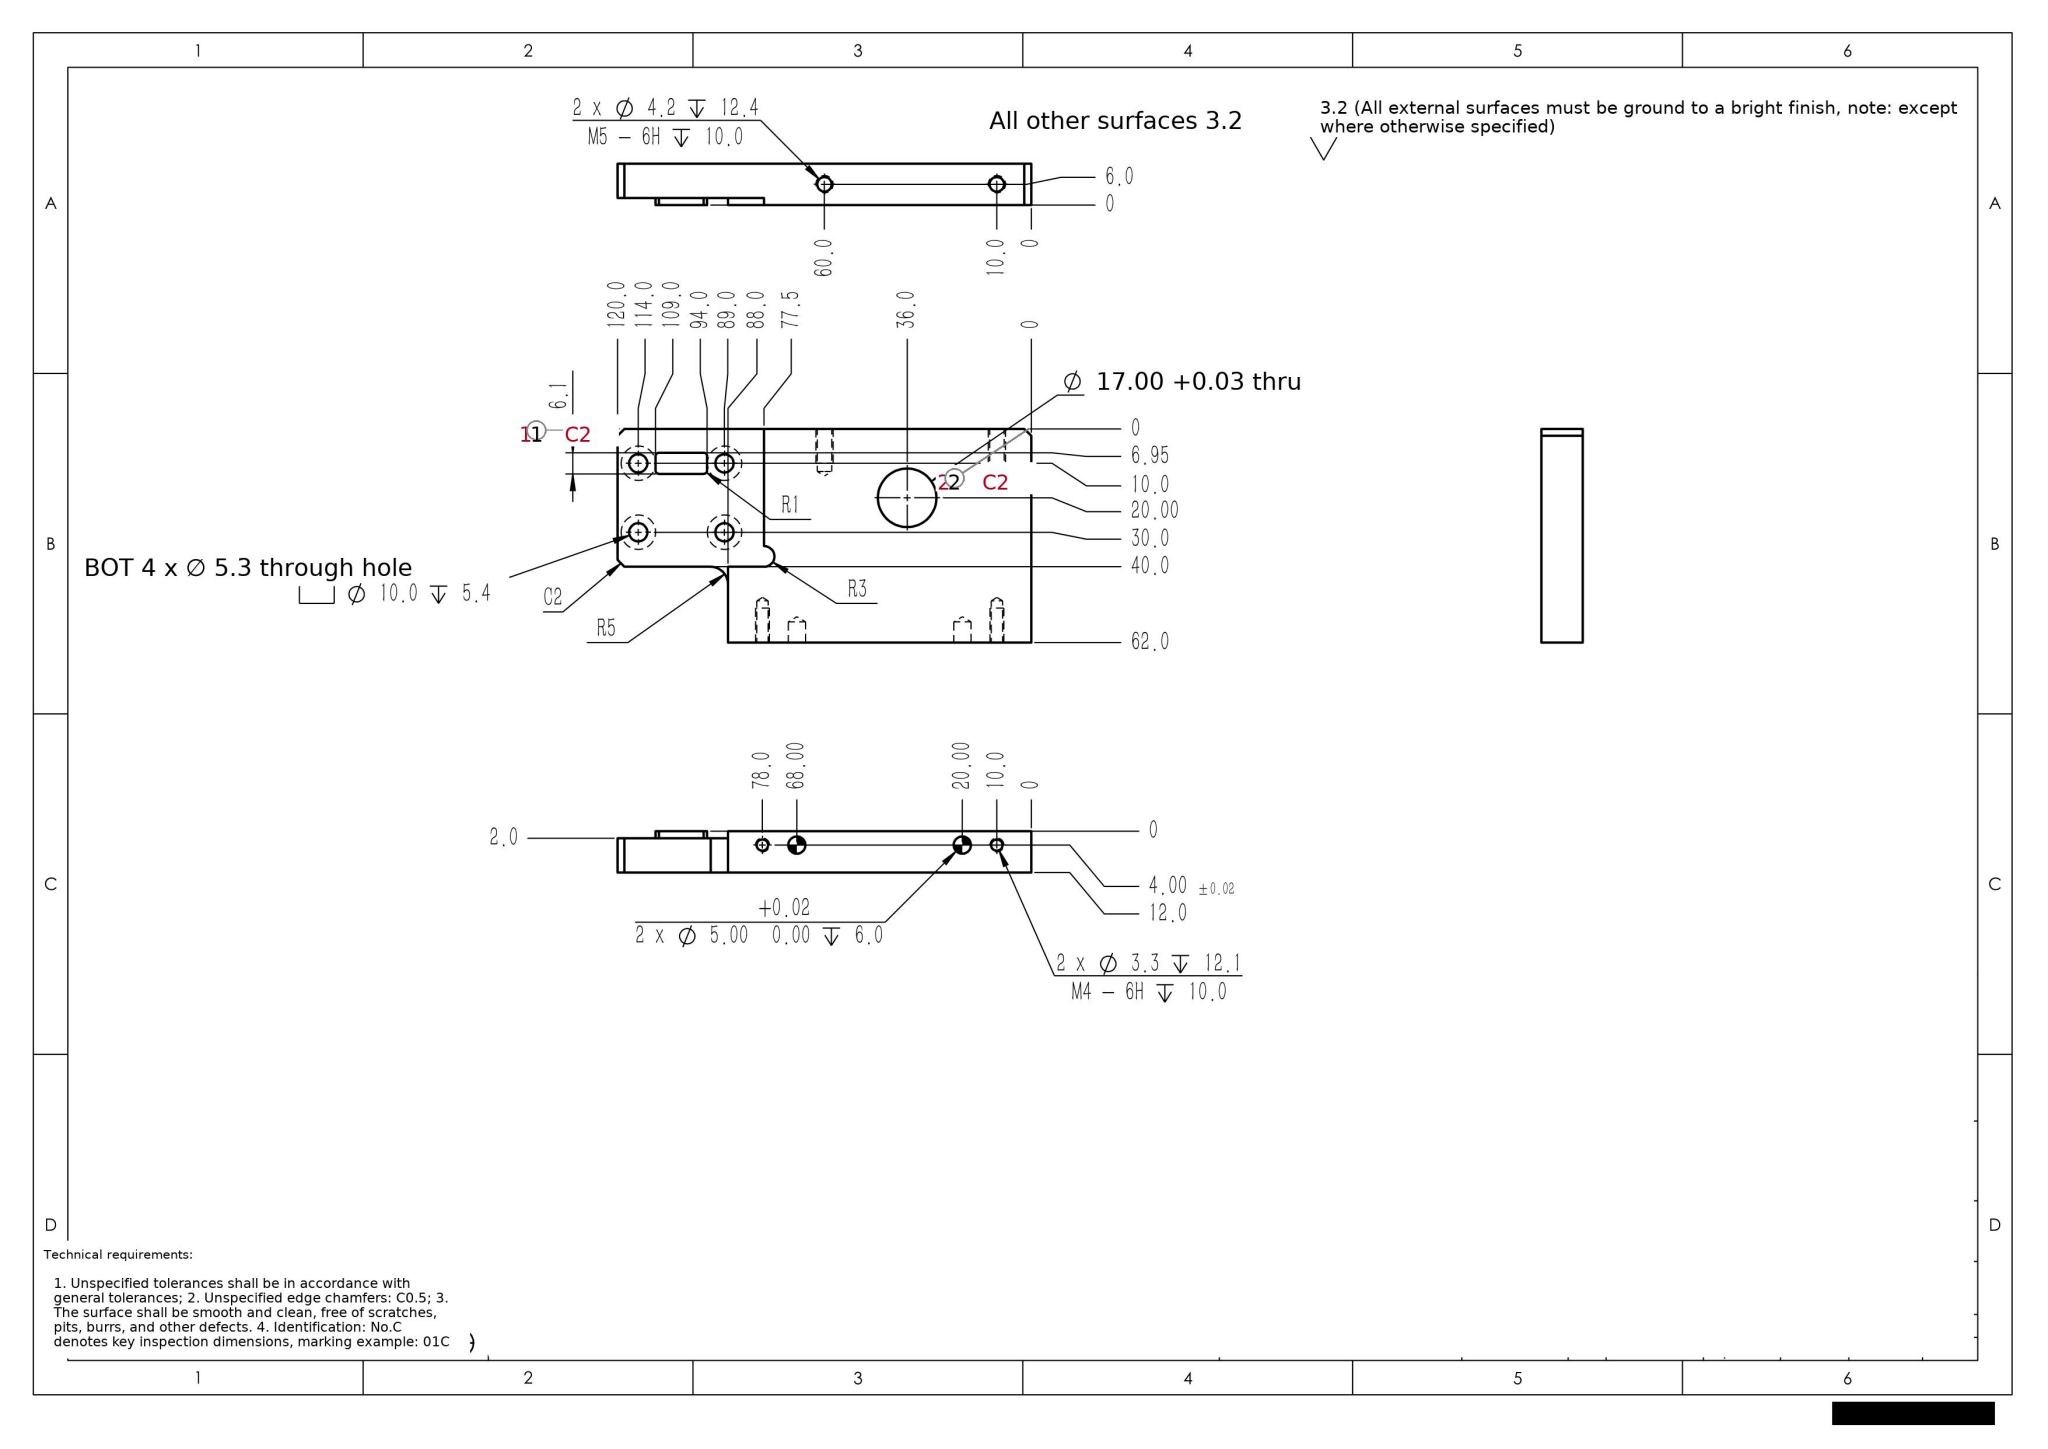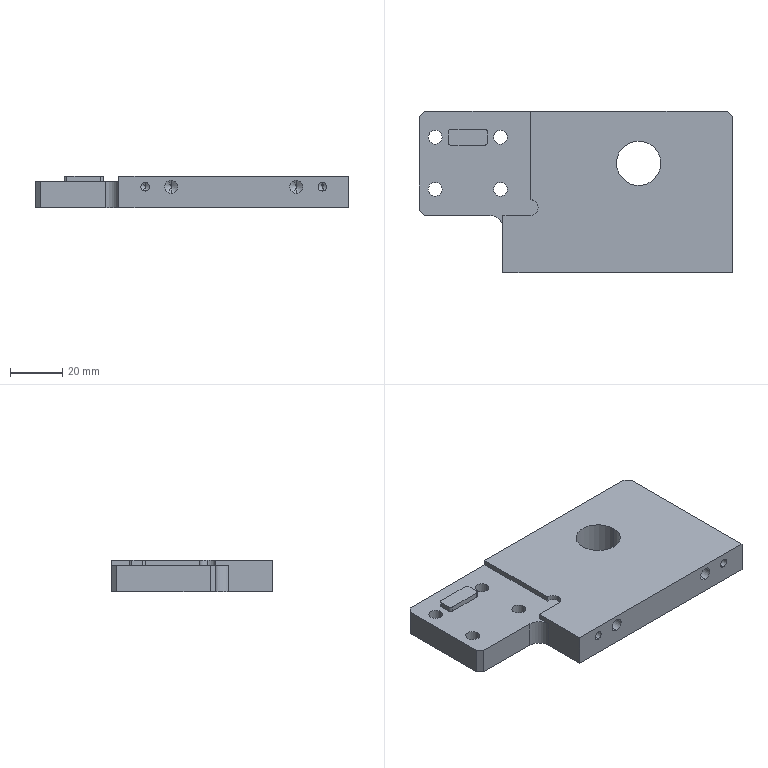Part | SolidWorks | mm | 1 solid | 72 faces | box 120 x 62 x 12 mm | volume 71925 mm3 | cylinder 37 | plane 23 | cone 12 | commonest cylinder face diameters 10 x9 5.3 x8 4.2 x4 5 x4 3.3 x4 2 x4 6 x2 17 x2
build123d program:
from build123d import *

# Parameters (mm, degrees)
SKETCH1_W                                       = 120
SKETCH1_H                                       = 40
BOSS_EXTRUDE1_DEPTH                             = 12
SKETCH2_R                                       = 8.5
CUT_EXTRUDE1_DEPTH                              = 65.374
SKETCH7_W                                       = 32
SKETCH7_H                                       = 2
CUT_EXTRUDE4_DEPTH                              = 74.103
M5_HEX_SOCKET_HEAD_CAP_SCREW_CBORE1_D           = 5.3
M5_HEX_SOCKET_HEAD_CAP_SCREW_CBORE1_CBORE_D     = 10
M5_HEX_SOCKET_HEAD_CAP_SCREW_CBORE1_CBORE_DEPTH = 5.4
SKETCH12_W                                      = 15
SKETCH12_H                                      = 6.1
BOSS_EXTRUDE2_DEPTH                             = 2
SKETCH13_W                                      = 88
SKETCH13_H                                      = 12
BOSS_EXTRUDE3_DEPTH                             = 22
M4_TAPPED_HOLE1_D                               = 3.3
M4_TAPPED_HOLE1_DEPTH                           = 12.1
M4_TAPPED_HOLE1_TIP                             = 0.9914
SIZE_MM_DOWEL_PIN_HOLE1_D                       = 5
SIZE_MM_DOWEL_PIN_HOLE1_DEPTH                   = 6
SIZE_MM_DOWEL_PIN_HOLE1_TIP                     = 1.502
M5_TAPPED_HOLE1_D                               = 4.2
M5_TAPPED_HOLE1_DEPTH                           = 12.4
M5_TAPPED_HOLE1_TIP                             = 1.262
SKETCH23_W                                      = 10.5
SKETCH23_H                                      = 40
CUT_EXTRUDE6_DEPTH                              = 2
FILLET3_R                                       = 5
FILLET2_R                                       = 1
CHAMFER1_SIZE                                   = 2
SKETCH24_R                                      = 3
CUT_EXTRUDE7_DEPTH                              = 2


with BuildPart() as part:
    # Sketch1 → Boss-Extrude1 (new body)
    with BuildSketch(Plane.XY):
        Rectangle(SKETCH1_W, SKETCH1_H)
    extrude(amount=BOSS_EXTRUDE1_DEPTH)

    # Sketch2 → Cut-Extrude1 (cut, through all)
    with BuildSketch(Plane.XY.offset(12)):
        with Locations((24, 0)):
            Circle(SKETCH2_R)
    extrude(amount=-CUT_EXTRUDE1_DEPTH, mode=Mode.SUBTRACT)

    # Sketch7 → Cut-Extrude4 (cut, through all)
    with BuildSketch(Plane(origin=(0, 20, 0), x_dir=(1, 0, 0), z_dir=(0, 1, 0))):
        with Locations((-44, -11)):
            Rectangle(SKETCH7_W, SKETCH7_H)
    extrude(amount=-CUT_EXTRUDE4_DEPTH, mode=Mode.SUBTRACT)

    # M5 Hex Socket Head Cap Screw CBORE1 (through all)
    with Locations(Plane(origin=(0, 0, 0), x_dir=(-1, 0, 0), z_dir=(0, 0, -1))):
        with Locations((54, -10), (29, -10), (29, 10), (54, 10)):
            CounterBoreHole(M5_HEX_SOCKET_HEAD_CAP_SCREW_CBORE1_D / 2, M5_HEX_SOCKET_HEAD_CAP_SCREW_CBORE1_CBORE_D / 2, M5_HEX_SOCKET_HEAD_CAP_SCREW_CBORE1_CBORE_DEPTH)

    # Sketch12 → Boss-Extrude2 (add)
    with BuildSketch(Plane.XY.offset(10)):
        with Locations((-41.5, 10)):
            Rectangle(SKETCH12_W, SKETCH12_H)
    extrude(amount=BOSS_EXTRUDE2_DEPTH)

    # Sketch13 → Boss-Extrude3 (add)
    with BuildSketch(Plane.XZ.offset(20)):
        with Locations((16, 6)):
            Rectangle(SKETCH13_W, SKETCH13_H)
    extrude(amount=BOSS_EXTRUDE3_DEPTH)

    # M4 Tapped Hole1
    with Locations(Plane(origin=(0, -42, 0), x_dir=(-1, 0, 0), z_dir=(0, -1, 0))):
        with Locations((18, -8), (-50, -8)):
            Hole(M4_TAPPED_HOLE1_D / 2, depth=M4_TAPPED_HOLE1_DEPTH)
            with Locations((0, 0, -(M4_TAPPED_HOLE1_DEPTH + M4_TAPPED_HOLE1_TIP / 2))):  # 118° drill point
                Cone(0, M4_TAPPED_HOLE1_D / 2, M4_TAPPED_HOLE1_TIP, mode=Mode.SUBTRACT)

    # Size mm Dowel Pin Hole1
    with Locations(Plane(origin=(0, -42, 0), x_dir=(-1, 0, 0), z_dir=(0, -1, 0))):
        with Locations((-40, -8), (8, -8)):
            Hole(SIZE_MM_DOWEL_PIN_HOLE1_D / 2, depth=SIZE_MM_DOWEL_PIN_HOLE1_DEPTH)
            with Locations((0, 0, -(SIZE_MM_DOWEL_PIN_HOLE1_DEPTH + SIZE_MM_DOWEL_PIN_HOLE1_TIP / 2))):  # 118° drill point
                Cone(0, SIZE_MM_DOWEL_PIN_HOLE1_D / 2, SIZE_MM_DOWEL_PIN_HOLE1_TIP, mode=Mode.SUBTRACT)

    # M5 Tapped Hole1
    with Locations(Plane(origin=(0, 20, 0), x_dir=(1, 0, 0), z_dir=(0, 1, 0))):
        with Locations((50, -6), (0, -6)):
            Hole(M5_TAPPED_HOLE1_D / 2, depth=M5_TAPPED_HOLE1_DEPTH)
            with Locations((0, 0, -(M5_TAPPED_HOLE1_DEPTH + M5_TAPPED_HOLE1_TIP / 2))):  # 118° drill point
                Cone(0, M5_TAPPED_HOLE1_D / 2, M5_TAPPED_HOLE1_TIP, mode=Mode.SUBTRACT)

    # Sketch23 → Cut-Extrude6 (cut)
    with BuildSketch(Plane.XY.offset(12)):
        with Locations((-22.75, 0)):
            Rectangle(SKETCH23_W, SKETCH23_H)
    extrude(amount=-CUT_EXTRUDE6_DEPTH, mode=Mode.SUBTRACT)

    # Fillet3
    fillet3_edges = [part.edges().sort_by_distance(p)[0] for p in [
        (-28, -20, 5),
    ]]
    fillet(fillet3_edges, radius=FILLET3_R)

    # Fillet2
    fillet2_edges = [part.edges().sort_by_distance(p)[0] for p in [
        (-49, 6.95, 11),
        (-49, 13.05, 11),
        (-34, 13.05, 11),
        (-34, 6.95, 11),
    ]]
    fillet(fillet2_edges, radius=FILLET2_R)

    # Chamfer1
    chamfer1_edges = [part.edges().sort_by_distance(p)[0] for p in [
        (-60, -20, 5),
        (-60, 20, 5),
        (60, 20, 6),
    ]]
    chamfer(chamfer1_edges, length=CHAMFER1_SIZE)

    # Sketch24 → Cut-Extrude7 (cut)
    with BuildSketch(Plane.XY.offset(12)):
        with Locations((-17.5, -17)):
            Circle(SKETCH24_R)
    extrude(amount=-CUT_EXTRUDE7_DEPTH, mode=Mode.SUBTRACT)


solid = part.part